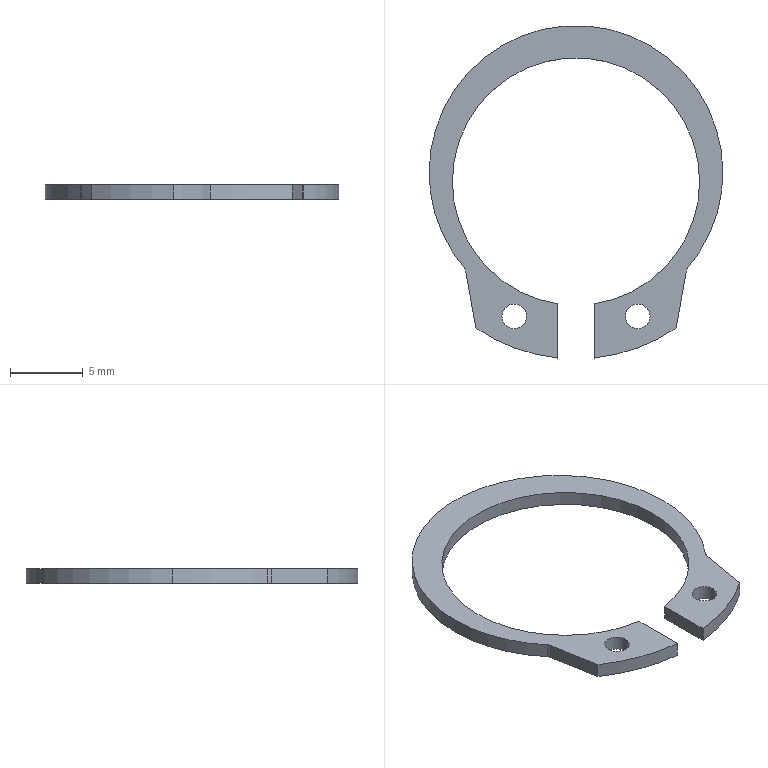Component | SolidWorks | 18A-typeShaftRetainingRing(GB-T894.1-1986)0-2 | 1 solid | 20 faces | box 20.2 x 22.86 x 1 mm | volume 122 mm3 | cylinder 14 | plane 6 | commonest cylinder face diameters 1.7 x4 20.2 x3 17 x3 24.4 x2 1 x2 | material 65Mn CH
build123d program:
from build123d import *

# Parameters (mm, degrees)
SKETCH1_R           = 0.85
BOSS_EXTRUDE1_DEPTH = 1


with BuildPart() as part:
    # Sketch1 → Boss-Extrude1 (new body)
    with BuildSketch(Plane.XY):
        with BuildLine():
            Line((-7.583, -6.16), (-6.894, -10.065))
            ThreePointArc((-6.894, -10.065), (-4.202, -11.454), (-1.25, -12.136))
            Line((-1.25, -12.136), (-1.25, -8.408))
            ThreePointArc((-1.25, -8.408), (0, 8.5), (1.25, -8.408))
            Line((1.25, -8.408), (1.25, -12.136))
            ThreePointArc((1.25, -12.136), (4.202, -11.454), (6.894, -10.065))
            Line((6.894, -10.065), (7.583, -6.16))
            ThreePointArc((7.583, -6.16), (7.623, -6.034), (7.694, -5.923))
            ThreePointArc((7.694, -5.923), (0, 10.72), (-7.694, -5.923))
            ThreePointArc((-7.694, -5.923), (-7.623, -6.034), (-7.583, -6.16))
        make_face()
        with Locations((-4.25, -9.27)):
            Circle(SKETCH1_R, mode=Mode.SUBTRACT)
        with Locations((4.25, -9.27)):
            Circle(SKETCH1_R, mode=Mode.SUBTRACT)
    extrude(amount=BOSS_EXTRUDE1_DEPTH)


solid = part.part

# Placed as in the assembly
solid = solid.moved(Location((-15.093, -37.782, 147.955), (0, 0, 0)))
STEP:
#1=COLOUR_RGB('',0.7922,0.8196,0.9333);
#2=FILL_AREA_STYLE_COLOUR('',#1);
#3=FILL_AREA_STYLE('',(#2));
#4=SURFACE_STYLE_FILL_AREA(#3);
#5=SURFACE_SIDE_STYLE('',(#4));
#6=SURFACE_STYLE_USAGE(.BOTH.,#5);
#7=PRESENTATION_STYLE_ASSIGNMENT((#6));
#8=CARTESIAN_POINT('',(-0.4604,-1.852,5.864));
#9=VERTEX_POINT('',#8);
#10=CARTESIAN_POINT('',(-0.3934,-1.852,5.864));
#11=VERTEX_POINT('',#10);
#12=CARTESIAN_POINT('',(-0.4269,-1.852,5.864));
#13=DIRECTION('',(0.,0.,1.));
#14=DIRECTION('',(1.,0.,0.));
#15=AXIS2_PLACEMENT_3D('',#12,#13,#14);
#16=CIRCLE('',#15,0.03346);
#17=EDGE_CURVE('',#9,#11,#16,.T.);
#18=ORIENTED_EDGE('',*,*,#17,.T.);
#19=CARTESIAN_POINT('',(-0.3934,-1.852,5.825));
#20=VERTEX_POINT('',#19);
#21=CARTESIAN_POINT('',(-0.3934,-1.852,5.864));
#22=DIRECTION('',(0.,0.,-1.));
#23=VECTOR('',#22,39.37);
#24=LINE('',#21,#23);
#25=EDGE_CURVE('',#11,#20,#24,.T.);
#26=ORIENTED_EDGE('',*,*,#25,.T.);
#27=CARTESIAN_POINT('',(-0.4604,-1.852,5.825));
#28=VERTEX_POINT('',#27);
#29=CARTESIAN_POINT('',(-0.4269,-1.852,5.825));
#30=DIRECTION('',(0.,0.,1.));
#31=DIRECTION('',(1.,0.,0.));
#32=AXIS2_PLACEMENT_3D('',#29,#30,#31);
#33=CIRCLE('',#32,0.03346);
#34=EDGE_CURVE('',#28,#20,#33,.T.);
#35=ORIENTED_EDGE('',*,*,#34,.F.);
#36=CARTESIAN_POINT('',(-0.4604,-1.852,5.864));
#37=DIRECTION('',(0.,0.,-1.));
#38=VECTOR('',#37,39.37);
#39=LINE('',#36,#38);
#40=EDGE_CURVE('',#9,#28,#39,.T.);
#41=ORIENTED_EDGE('',*,*,#40,.F.);
#42=EDGE_LOOP('',(#18,#26,#35,#41));
#43=FACE_OUTER_BOUND('',#42,.T.);
#44=CARTESIAN_POINT('',(-0.4269,-1.852,5.864));
#45=DIRECTION('',(0.,0.,-1.));
#46=DIRECTION('',(-1.,0.,0.));
#47=AXIS2_PLACEMENT_3D('',#44,#45,#46);
#48=CYLINDRICAL_SURFACE('',#47,0.03346);
#49=ADVANCED_FACE('',(#43),#48,.F.);
#50=CARTESIAN_POINT('',(-0.795,-1.852,5.864));
#51=VERTEX_POINT('',#50);
#52=CARTESIAN_POINT('',(-0.7281,-1.852,5.864));
#53=VERTEX_POINT('',#52);
#54=CARTESIAN_POINT('',(-0.7615,-1.852,5.864));
#55=DIRECTION('',(0.,0.,1.));
#56=DIRECTION('',(1.,0.,0.));
#57=AXIS2_PLACEMENT_3D('',#54,#55,#56);
#58=CIRCLE('',#57,0.03346);
#59=EDGE_CURVE('',#51,#53,#58,.T.);
#60=ORIENTED_EDGE('',*,*,#59,.T.);
#61=CARTESIAN_POINT('',(-0.7281,-1.852,5.825));
#62=VERTEX_POINT('',#61);
#63=CARTESIAN_POINT('',(-0.7281,-1.852,5.864));
#64=DIRECTION('',(0.,0.,-1.));
#65=VECTOR('',#64,39.37);
#66=LINE('',#63,#65);
#67=EDGE_CURVE('',#53,#62,#66,.T.);
#68=ORIENTED_EDGE('',*,*,#67,.T.);
#69=CARTESIAN_POINT('',(-0.795,-1.852,5.825));
#70=VERTEX_POINT('',#69);
#71=CARTESIAN_POINT('',(-0.7615,-1.852,5.825));
#72=DIRECTION('',(0.,0.,1.));
#73=DIRECTION('',(1.,0.,0.));
#74=AXIS2_PLACEMENT_3D('',#71,#72,#73);
#75=CIRCLE('',#74,0.03346);
#76=EDGE_CURVE('',#70,#62,#75,.T.);
#77=ORIENTED_EDGE('',*,*,#76,.F.);
#78=CARTESIAN_POINT('',(-0.795,-1.852,5.864));
#79=DIRECTION('',(0.,0.,-1.));
#80=VECTOR('',#79,39.37);
#81=LINE('',#78,#80);
#82=EDGE_CURVE('',#51,#70,#81,.T.);
#83=ORIENTED_EDGE('',*,*,#82,.F.);
#84=EDGE_LOOP('',(#60,#68,#77,#83));
#85=FACE_OUTER_BOUND('',#84,.T.);
#86=CARTESIAN_POINT('',(-0.7615,-1.852,5.864));
#87=DIRECTION('',(0.,0.,-1.));
#88=DIRECTION('',(-1.,0.,0.));
#89=AXIS2_PLACEMENT_3D('',#86,#87,#88);
#90=CYLINDRICAL_SURFACE('',#89,0.03346);
#91=ADVANCED_FACE('',(#85),#90,.F.);
#92=CARTESIAN_POINT('',(-0.1966,-1.463,5.864));
#93=VERTEX_POINT('',#92);
#94=CARTESIAN_POINT('',(-0.9919,-1.463,5.864));
#95=VERTEX_POINT('',#94);
#96=CARTESIAN_POINT('',(-0.5942,-1.463,5.864));
#97=DIRECTION('',(0.,0.,1.));
#98=DIRECTION('',(1.,0.,0.));
#99=AXIS2_PLACEMENT_3D('',#96,#97,#98);
#100=CIRCLE('',#99,0.3976);
#101=EDGE_CURVE('',#93,#95,#100,.T.);
#102=ORIENTED_EDGE('',*,*,#101,.F.);
#103=CARTESIAN_POINT('',(-0.1966,-1.463,5.825));
#104=VERTEX_POINT('',#103);
#105=CARTESIAN_POINT('',(-0.1966,-1.463,5.864));
#106=DIRECTION('',(0.,0.,-1.));
#107=VECTOR('',#106,39.37);
#108=LINE('',#105,#107);
#109=EDGE_CURVE('',#93,#104,#108,.T.);
#110=ORIENTED_EDGE('',*,*,#109,.T.);
#111=CARTESIAN_POINT('',(-0.9919,-1.463,5.825));
#112=VERTEX_POINT('',#111);
#113=CARTESIAN_POINT('',(-0.5942,-1.463,5.825));
#114=DIRECTION('',(0.,0.,1.));
#115=DIRECTION('',(1.,0.,0.));
#116=AXIS2_PLACEMENT_3D('',#113,#114,#115);
#117=CIRCLE('',#116,0.3976);
#118=EDGE_CURVE('',#104,#112,#117,.T.);
#119=ORIENTED_EDGE('',*,*,#118,.T.);
#120=CARTESIAN_POINT('',(-0.9919,-1.463,5.864));
#121=DIRECTION('',(0.,0.,-1.));
#122=VECTOR('',#121,39.37);
#123=LINE('',#120,#122);
#124=EDGE_CURVE('',#95,#112,#123,.T.);
#125=ORIENTED_EDGE('',*,*,#124,.F.);
#126=EDGE_LOOP('',(#102,#110,#119,#125));
#127=FACE_OUTER_BOUND('',#126,.T.);
#128=CARTESIAN_POINT('',(-0.5942,-1.463,5.864));
#129=DIRECTION('',(0.,0.,-1.));
#130=DIRECTION('',(-1.,0.,0.));
#131=AXIS2_PLACEMENT_3D('',#128,#129,#130);
#132=CYLINDRICAL_SURFACE('',#131,0.3976);
#133=ADVANCED_FACE('',(#127),#132,.T.);
#134=CARTESIAN_POINT('',(-0.8971,-1.721,5.864));
#135=VERTEX_POINT('',#134);
#136=CARTESIAN_POINT('',(-0.5942,-1.463,5.864));
#137=DIRECTION('',(0.,0.,1.));
#138=DIRECTION('',(1.,0.,0.));
#139=AXIS2_PLACEMENT_3D('',#136,#137,#138);
#140=CIRCLE('',#139,0.3976);
#141=EDGE_CURVE('',#95,#135,#140,.T.);
#142=ORIENTED_EDGE('',*,*,#141,.F.);
#143=ORIENTED_EDGE('',*,*,#124,.T.);
#144=CARTESIAN_POINT('',(-0.8971,-1.721,5.825));
#145=VERTEX_POINT('',#144);
#146=CARTESIAN_POINT('',(-0.5942,-1.463,5.825));
#147=DIRECTION('',(0.,0.,1.));
#148=DIRECTION('',(1.,0.,0.));
#149=AXIS2_PLACEMENT_3D('',#146,#147,#148);
#150=CIRCLE('',#149,0.3976);
#151=EDGE_CURVE('',#112,#145,#150,.T.);
#152=ORIENTED_EDGE('',*,*,#151,.T.);
#153=CARTESIAN_POINT('',(-0.8971,-1.721,5.864));
#154=DIRECTION('',(0.,0.,-1.));
#155=VECTOR('',#154,39.37);
#156=LINE('',#153,#155);
#157=EDGE_CURVE('',#135,#145,#156,.T.);
#158=ORIENTED_EDGE('',*,*,#157,.F.);
#159=EDGE_LOOP('',(#142,#143,#152,#158));
#160=FACE_OUTER_BOUND('',#159,.T.);
#161=CARTESIAN_POINT('',(-0.5942,-1.463,5.864));
#162=DIRECTION('',(0.,0.,-1.));
#163=DIRECTION('',(-1.,0.,0.));
#164=AXIS2_PLACEMENT_3D('',#161,#162,#163);
#165=CYLINDRICAL_SURFACE('',#164,0.3976);
#166=ADVANCED_FACE('',(#160),#165,.T.);
#167=CARTESIAN_POINT('',(-0.2596,-1.487,5.864));
#168=VERTEX_POINT('',#167);
#169=CARTESIAN_POINT('',(-0.545,-1.818,5.864));
#170=VERTEX_POINT('',#169);
#171=CARTESIAN_POINT('',(-0.5942,-1.487,5.864));
#172=DIRECTION('',(0.,0.,-1.));
#173=DIRECTION('',(1.,0.,0.));
#174=AXIS2_PLACEMENT_3D('',#171,#172,#173);
#175=CIRCLE('',#174,0.3346);
#176=EDGE_CURVE('',#168,#170,#175,.T.);
#177=ORIENTED_EDGE('',*,*,#176,.F.);
#178=CARTESIAN_POINT('',(-0.2596,-1.487,5.825));
#179=VERTEX_POINT('',#178);
#180=CARTESIAN_POINT('',(-0.2596,-1.487,5.864));
#181=DIRECTION('',(0.,0.,-1.));
#182=VECTOR('',#181,39.37);
#183=LINE('',#180,#182);
#184=EDGE_CURVE('',#168,#179,#183,.T.);
#185=ORIENTED_EDGE('',*,*,#184,.T.);
#186=CARTESIAN_POINT('',(-0.545,-1.818,5.825));
#187=VERTEX_POINT('',#186);
#188=CARTESIAN_POINT('',(-0.5942,-1.487,5.825));
#189=DIRECTION('',(0.,0.,-1.));
#190=DIRECTION('',(1.,0.,0.));
#191=AXIS2_PLACEMENT_3D('',#188,#189,#190);
#192=CIRCLE('',#191,0.3346);
#193=EDGE_CURVE('',#179,#187,#192,.T.);
#194=ORIENTED_EDGE('',*,*,#193,.T.);
#195=CARTESIAN_POINT('',(-0.545,-1.818,5.864));
#196=DIRECTION('',(0.,0.,-1.));
#197=VECTOR('',#196,39.37);
#198=LINE('',#195,#197);
#199=EDGE_CURVE('',#170,#187,#198,.T.);
#200=ORIENTED_EDGE('',*,*,#199,.F.);
#201=EDGE_LOOP('',(#177,#185,#194,#200));
#202=FACE_OUTER_BOUND('',#201,.T.);
#203=CARTESIAN_POINT('',(-0.5942,-1.487,5.864));
#204=DIRECTION('',(0.,0.,-1.));
#205=DIRECTION('',(-1.,0.,0.));
#206=AXIS2_PLACEMENT_3D('',#203,#204,#205);
#207=CYLINDRICAL_SURFACE('',#206,0.3346);
#208=ADVANCED_FACE('',(#202),#207,.F.);
#209=ORIENTED_EDGE('',*,*,#184,.F.);
#210=CARTESIAN_POINT('',(-0.9289,-1.487,5.864));
#211=VERTEX_POINT('',#210);
#212=CARTESIAN_POINT('',(-0.5942,-1.487,5.864));
#213=DIRECTION('',(0.,0.,-1.));
#214=DIRECTION('',(1.,0.,0.));
#215=AXIS2_PLACEMENT_3D('',#212,#213,#214);
#216=CIRCLE('',#215,0.3346);
#217=EDGE_CURVE('',#211,#168,#216,.T.);
#218=ORIENTED_EDGE('',*,*,#217,.F.);
#219=CARTESIAN_POINT('',(-0.9289,-1.487,5.825));
#220=VERTEX_POINT('',#219);
#221=CARTESIAN_POINT('',(-0.9289,-1.487,5.864));
#222=DIRECTION('',(0.,0.,-1.));
#223=VECTOR('',#222,39.37);
#224=LINE('',#221,#223);
#225=EDGE_CURVE('',#211,#220,#224,.T.);
#226=ORIENTED_EDGE('',*,*,#225,.T.);
#227=CARTESIAN_POINT('',(-0.5942,-1.487,5.825));
#228=DIRECTION('',(0.,0.,-1.));
#229=DIRECTION('',(1.,0.,0.));
#230=AXIS2_PLACEMENT_3D('',#227,#228,#229);
#231=CIRCLE('',#230,0.3346);
#232=EDGE_CURVE('',#220,#179,#231,.T.);
#233=ORIENTED_EDGE('',*,*,#232,.T.);
#234=EDGE_LOOP('',(#209,#218,#226,#233));
#235=FACE_OUTER_BOUND('',#234,.T.);
#236=CARTESIAN_POINT('',(-0.5942,-1.487,5.864));
#237=DIRECTION('',(0.,0.,-1.));
#238=DIRECTION('',(-1.,0.,0.));
#239=AXIS2_PLACEMENT_3D('',#236,#237,#238);
#240=CYLINDRICAL_SURFACE('',#239,0.3346);
#241=ADVANCED_FACE('',(#235),#240,.F.);
#242=ORIENTED_EDGE('',*,*,#59,.F.);
#243=CARTESIAN_POINT('',(-0.7615,-1.852,5.864));
#244=DIRECTION('',(0.,0.,1.));
#245=DIRECTION('',(1.,0.,0.));
#246=AXIS2_PLACEMENT_3D('',#243,#244,#245);
#247=CIRCLE('',#246,0.03346);
#248=EDGE_CURVE('',#53,#51,#247,.T.);
#249=ORIENTED_EDGE('',*,*,#248,.F.);
#250=EDGE_LOOP('',(#242,#249));
#251=FACE_BOUND('',#250,.T.);
#252=CARTESIAN_POINT('',(-0.6434,-1.818,5.864));
#253=VERTEX_POINT('',#252);
#254=CARTESIAN_POINT('',(-0.5942,-1.487,5.864));
#255=DIRECTION('',(0.,0.,-1.));
#256=DIRECTION('',(1.,0.,0.));
#257=AXIS2_PLACEMENT_3D('',#254,#255,#256);
#258=CIRCLE('',#257,0.3346);
#259=EDGE_CURVE('',#253,#211,#258,.T.);
#260=ORIENTED_EDGE('',*,*,#259,.T.);
#261=ORIENTED_EDGE('',*,*,#217,.T.);
#262=ORIENTED_EDGE('',*,*,#176,.T.);
#263=CARTESIAN_POINT('',(-0.545,-1.965,5.864));
#264=VERTEX_POINT('',#263);
#265=CARTESIAN_POINT('',(-0.545,-1.818,5.864));
#266=DIRECTION('',(0.,-1.,0.));
#267=VECTOR('',#266,39.37);
#268=LINE('',#265,#267);
#269=EDGE_CURVE('',#170,#264,#268,.T.);
#270=ORIENTED_EDGE('',*,*,#269,.T.);
#271=CARTESIAN_POINT('',(-0.3228,-1.884,5.864));
#272=VERTEX_POINT('',#271);
#273=CARTESIAN_POINT('',(-0.5942,-1.487,5.864));
#274=DIRECTION('',(0.,0.,1.));
#275=DIRECTION('',(1.,0.,0.));
#276=AXIS2_PLACEMENT_3D('',#273,#274,#275);
#277=CIRCLE('',#276,0.4803);
#278=EDGE_CURVE('',#264,#272,#277,.T.);
#279=ORIENTED_EDGE('',*,*,#278,.T.);
#280=CARTESIAN_POINT('',(-0.2957,-1.73,5.864));
#281=VERTEX_POINT('',#280);
#282=CARTESIAN_POINT('',(-0.2957,-1.73,5.864));
#283=DIRECTION('',(0.1736,0.9848,0.));
#284=VECTOR('',#283,39.37);
#285=LINE('',#282,#284);
#286=EDGE_CURVE('',#272,#281,#285,.T.);
#287=ORIENTED_EDGE('',*,*,#286,.T.);
#288=CARTESIAN_POINT('',(-0.2913,-1.721,5.864));
#289=VERTEX_POINT('',#288);
#290=CARTESIAN_POINT('',(-0.2763,-1.733,5.864));
#291=DIRECTION('',(0.,0.,-1.));
#292=DIRECTION('',(1.,0.,0.));
#293=AXIS2_PLACEMENT_3D('',#290,#291,#292);
#294=CIRCLE('',#293,0.01969);
#295=EDGE_CURVE('',#281,#289,#294,.T.);
#296=ORIENTED_EDGE('',*,*,#295,.T.);
#297=CARTESIAN_POINT('',(-0.5942,-1.463,5.864));
#298=DIRECTION('',(0.,0.,1.));
#299=DIRECTION('',(1.,0.,0.));
#300=AXIS2_PLACEMENT_3D('',#297,#298,#299);
#301=CIRCLE('',#300,0.3976);
#302=EDGE_CURVE('',#289,#93,#301,.T.);
#303=ORIENTED_EDGE('',*,*,#302,.T.);
#304=ORIENTED_EDGE('',*,*,#101,.T.);
#305=ORIENTED_EDGE('',*,*,#141,.T.);
#306=CARTESIAN_POINT('',(-0.8927,-1.73,5.864));
#307=VERTEX_POINT('',#306);
#308=CARTESIAN_POINT('',(-0.9121,-1.733,5.864));
#309=DIRECTION('',(0.,0.,-1.));
#310=DIRECTION('',(1.,0.,0.));
#311=AXIS2_PLACEMENT_3D('',#308,#309,#310);
#312=CIRCLE('',#311,0.01969);
#313=EDGE_CURVE('',#135,#307,#312,.T.);
#314=ORIENTED_EDGE('',*,*,#313,.T.);
#315=CARTESIAN_POINT('',(-0.8656,-1.884,5.864));
#316=VERTEX_POINT('',#315);
#317=CARTESIAN_POINT('',(-0.8927,-1.73,5.864));
#318=DIRECTION('',(0.1736,-0.9848,0.));
#319=VECTOR('',#318,39.37);
#320=LINE('',#317,#319);
#321=EDGE_CURVE('',#307,#316,#320,.T.);
#322=ORIENTED_EDGE('',*,*,#321,.T.);
#323=CARTESIAN_POINT('',(-0.6434,-1.965,5.864));
#324=VERTEX_POINT('',#323);
#325=CARTESIAN_POINT('',(-0.5942,-1.487,5.864));
#326=DIRECTION('',(0.,0.,1.));
#327=DIRECTION('',(1.,0.,0.));
#328=AXIS2_PLACEMENT_3D('',#325,#326,#327);
#329=CIRCLE('',#328,0.4803);
#330=EDGE_CURVE('',#316,#324,#329,.T.);
#331=ORIENTED_EDGE('',*,*,#330,.T.);
#332=CARTESIAN_POINT('',(-0.6434,-1.818,5.864));
#333=DIRECTION('',(0.,1.,0.));
#334=VECTOR('',#333,39.37);
#335=LINE('',#332,#334);
#336=EDGE_CURVE('',#324,#253,#335,.T.);
#337=ORIENTED_EDGE('',*,*,#336,.T.);
#338=EDGE_LOOP('',(#260,#261,#262,#270,#279,#287,#296,#303,#304,#305,#314,#322,#331,#337));
#339=FACE_OUTER_BOUND('',#338,.T.);
#340=ORIENTED_EDGE('',*,*,#17,.F.);
#341=CARTESIAN_POINT('',(-0.4269,-1.852,5.864));
#342=DIRECTION('',(0.,0.,1.));
#343=DIRECTION('',(1.,0.,0.));
#344=AXIS2_PLACEMENT_3D('',#341,#342,#343);
#345=CIRCLE('',#344,0.03346);
#346=EDGE_CURVE('',#11,#9,#345,.T.);
#347=ORIENTED_EDGE('',*,*,#346,.F.);
#348=EDGE_LOOP('',(#340,#347));
#349=FACE_BOUND('',#348,.T.);
#350=CARTESIAN_POINT('',(-0.5942,-1.487,5.864));
#351=DIRECTION('',(0.,0.,1.));
#352=DIRECTION('',(1.,0.,0.));
#353=AXIS2_PLACEMENT_3D('',#350,#351,#352);
#354=PLANE('',#353);
#355=ADVANCED_FACE('',(#251,#339,#349),#354,.T.);
#356=CARTESIAN_POINT('',(-0.6434,-1.818,5.825));
#357=VERTEX_POINT('',#356);
#358=CARTESIAN_POINT('',(-0.5942,-1.487,5.825));
#359=DIRECTION('',(0.,0.,-1.));
#360=DIRECTION('',(1.,0.,0.));
#361=AXIS2_PLACEMENT_3D('',#358,#359,#360);
#362=CIRCLE('',#361,0.3346);
#363=EDGE_CURVE('',#357,#220,#362,.T.);
#364=ORIENTED_EDGE('',*,*,#363,.F.);
#365=CARTESIAN_POINT('',(-0.6434,-1.965,5.825));
#366=VERTEX_POINT('',#365);
#367=CARTESIAN_POINT('',(-0.6434,-1.818,5.825));
#368=DIRECTION('',(0.,1.,0.));
#369=VECTOR('',#368,39.37);
#370=LINE('',#367,#369);
#371=EDGE_CURVE('',#366,#357,#370,.T.);
#372=ORIENTED_EDGE('',*,*,#371,.F.);
#373=CARTESIAN_POINT('',(-0.8656,-1.884,5.825));
#374=VERTEX_POINT('',#373);
#375=CARTESIAN_POINT('',(-0.5942,-1.487,5.825));
#376=DIRECTION('',(0.,0.,1.));
#377=DIRECTION('',(1.,0.,0.));
#378=AXIS2_PLACEMENT_3D('',#375,#376,#377);
#379=CIRCLE('',#378,0.4803);
#380=EDGE_CURVE('',#374,#366,#379,.T.);
#381=ORIENTED_EDGE('',*,*,#380,.F.);
#382=CARTESIAN_POINT('',(-0.8927,-1.73,5.825));
#383=VERTEX_POINT('',#382);
#384=CARTESIAN_POINT('',(-0.8927,-1.73,5.825));
#385=DIRECTION('',(0.1736,-0.9848,0.));
#386=VECTOR('',#385,39.37);
#387=LINE('',#384,#386);
#388=EDGE_CURVE('',#383,#374,#387,.T.);
#389=ORIENTED_EDGE('',*,*,#388,.F.);
#390=CARTESIAN_POINT('',(-0.9121,-1.733,5.825));
#391=DIRECTION('',(0.,0.,-1.));
#392=DIRECTION('',(1.,0.,0.));
#393=AXIS2_PLACEMENT_3D('',#390,#391,#392);
#394=CIRCLE('',#393,0.01969);
#395=EDGE_CURVE('',#145,#383,#394,.T.);
#396=ORIENTED_EDGE('',*,*,#395,.F.);
#397=ORIENTED_EDGE('',*,*,#151,.F.);
#398=ORIENTED_EDGE('',*,*,#118,.F.);
#399=CARTESIAN_POINT('',(-0.2913,-1.721,5.825));
#400=VERTEX_POINT('',#399);
#401=CARTESIAN_POINT('',(-0.5942,-1.463,5.825));
#402=DIRECTION('',(0.,0.,1.));
#403=DIRECTION('',(1.,0.,0.));
#404=AXIS2_PLACEMENT_3D('',#401,#402,#403);
#405=CIRCLE('',#404,0.3976);
#406=EDGE_CURVE('',#400,#104,#405,.T.);
#407=ORIENTED_EDGE('',*,*,#406,.F.);
#408=CARTESIAN_POINT('',(-0.2957,-1.73,5.825));
#409=VERTEX_POINT('',#408);
#410=CARTESIAN_POINT('',(-0.2763,-1.733,5.825));
#411=DIRECTION('',(0.,0.,-1.));
#412=DIRECTION('',(1.,0.,0.));
#413=AXIS2_PLACEMENT_3D('',#410,#411,#412);
#414=CIRCLE('',#413,0.01969);
#415=EDGE_CURVE('',#409,#400,#414,.T.);
#416=ORIENTED_EDGE('',*,*,#415,.F.);
#417=CARTESIAN_POINT('',(-0.3228,-1.884,5.825));
#418=VERTEX_POINT('',#417);
#419=CARTESIAN_POINT('',(-0.2957,-1.73,5.825));
#420=DIRECTION('',(0.1736,0.9848,0.));
#421=VECTOR('',#420,39.37);
#422=LINE('',#419,#421);
#423=EDGE_CURVE('',#418,#409,#422,.T.);
#424=ORIENTED_EDGE('',*,*,#423,.F.);
#425=CARTESIAN_POINT('',(-0.545,-1.965,5.825));
#426=VERTEX_POINT('',#425);
#427=CARTESIAN_POINT('',(-0.5942,-1.487,5.825));
#428=DIRECTION('',(0.,0.,1.));
#429=DIRECTION('',(1.,0.,0.));
#430=AXIS2_PLACEMENT_3D('',#427,#428,#429);
#431=CIRCLE('',#430,0.4803);
#432=EDGE_CURVE('',#426,#418,#431,.T.);
#433=ORIENTED_EDGE('',*,*,#432,.F.);
#434=CARTESIAN_POINT('',(-0.545,-1.818,5.825));
#435=DIRECTION('',(0.,-1.,0.));
#436=VECTOR('',#435,39.37);
#437=LINE('',#434,#436);
#438=EDGE_CURVE('',#187,#426,#437,.T.);
#439=ORIENTED_EDGE('',*,*,#438,.F.);
#440=ORIENTED_EDGE('',*,*,#193,.F.);
#441=ORIENTED_EDGE('',*,*,#232,.F.);
#442=EDGE_LOOP('',(#364,#372,#381,#389,#396,#397,#398,#407,#416,#424,#433,#439,#440,#441));
#443=FACE_OUTER_BOUND('',#442,.T.);
#444=ORIENTED_EDGE('',*,*,#76,.T.);
#445=CARTESIAN_POINT('',(-0.7615,-1.852,5.825));
#446=DIRECTION('',(0.,0.,1.));
#447=DIRECTION('',(1.,0.,0.));
#448=AXIS2_PLACEMENT_3D('',#445,#446,#447);
#449=CIRCLE('',#448,0.03346);
#450=EDGE_CURVE('',#62,#70,#449,.T.);
#451=ORIENTED_EDGE('',*,*,#450,.T.);
#452=EDGE_LOOP('',(#444,#451));
#453=FACE_BOUND('',#452,.T.);
#454=ORIENTED_EDGE('',*,*,#34,.T.);
#455=CARTESIAN_POINT('',(-0.4269,-1.852,5.825));
#456=DIRECTION('',(0.,0.,1.));
#457=DIRECTION('',(1.,0.,0.));
#458=AXIS2_PLACEMENT_3D('',#455,#456,#457);
#459=CIRCLE('',#458,0.03346);
#460=EDGE_CURVE('',#20,#28,#459,.T.);
#461=ORIENTED_EDGE('',*,*,#460,.T.);
#462=EDGE_LOOP('',(#454,#461));
#463=FACE_BOUND('',#462,.T.);
#464=CARTESIAN_POINT('',(-0.5942,-1.487,5.825));
#465=DIRECTION('',(0.,0.,1.));
#466=DIRECTION('',(1.,0.,0.));
#467=AXIS2_PLACEMENT_3D('',#464,#465,#466);
#468=PLANE('',#467);
#469=ADVANCED_FACE('',(#443,#453,#463),#468,.F.);
#470=ORIENTED_EDGE('',*,*,#225,.F.);
#471=ORIENTED_EDGE('',*,*,#259,.F.);
#472=CARTESIAN_POINT('',(-0.6434,-1.818,5.864));
#473=DIRECTION('',(0.,0.,-1.));
#474=VECTOR('',#473,39.37);
#475=LINE('',#472,#474);
#476=EDGE_CURVE('',#253,#357,#475,.T.);
#477=ORIENTED_EDGE('',*,*,#476,.T.);
#478=ORIENTED_EDGE('',*,*,#363,.T.);
#479=EDGE_LOOP('',(#470,#471,#477,#478));
#480=FACE_OUTER_BOUND('',#479,.T.);
#481=CARTESIAN_POINT('',(-0.5942,-1.487,5.864));
#482=DIRECTION('',(0.,0.,-1.));
#483=DIRECTION('',(-1.,0.,0.));
#484=AXIS2_PLACEMENT_3D('',#481,#482,#483);
#485=CYLINDRICAL_SURFACE('',#484,0.3346);
#486=ADVANCED_FACE('',(#480),#485,.F.);
#487=ORIENTED_EDGE('',*,*,#438,.T.);
#488=CARTESIAN_POINT('',(-0.545,-1.965,5.864));
#489=DIRECTION('',(0.,0.,-1.));
#490=VECTOR('',#489,39.37);
#491=LINE('',#488,#490);
#492=EDGE_CURVE('',#264,#426,#491,.T.);
#493=ORIENTED_EDGE('',*,*,#492,.F.);
#494=ORIENTED_EDGE('',*,*,#269,.F.);
#495=ORIENTED_EDGE('',*,*,#199,.T.);
#496=EDGE_LOOP('',(#487,#493,#494,#495));
#497=FACE_OUTER_BOUND('',#496,.T.);
#498=CARTESIAN_POINT('',(-0.545,-1.818,5.864));
#499=DIRECTION('',(1.,0.,0.));
#500=DIRECTION('',(0.,0.,-1.));
#501=AXIS2_PLACEMENT_3D('',#498,#499,#500);
#502=PLANE('',#501);
#503=ADVANCED_FACE('',(#497),#502,.F.);
#504=ORIENTED_EDGE('',*,*,#432,.T.);
#505=CARTESIAN_POINT('',(-0.3228,-1.884,5.864));
#506=DIRECTION('',(0.,0.,-1.));
#507=VECTOR('',#506,39.37);
#508=LINE('',#505,#507);
#509=EDGE_CURVE('',#272,#418,#508,.T.);
#510=ORIENTED_EDGE('',*,*,#509,.F.);
#511=ORIENTED_EDGE('',*,*,#278,.F.);
#512=ORIENTED_EDGE('',*,*,#492,.T.);
#513=EDGE_LOOP('',(#504,#510,#511,#512));
#514=FACE_OUTER_BOUND('',#513,.T.);
#515=CARTESIAN_POINT('',(-0.5942,-1.487,5.864));
#516=DIRECTION('',(0.,0.,-1.));
#517=DIRECTION('',(-1.,0.,0.));
#518=AXIS2_PLACEMENT_3D('',#515,#516,#517);
#519=CYLINDRICAL_SURFACE('',#518,0.4803);
#520=ADVANCED_FACE('',(#514),#519,.T.);
#521=ORIENTED_EDGE('',*,*,#423,.T.);
#522=CARTESIAN_POINT('',(-0.2957,-1.73,5.864));
#523=DIRECTION('',(0.,0.,-1.));
#524=VECTOR('',#523,39.37);
#525=LINE('',#522,#524);
#526=EDGE_CURVE('',#281,#409,#525,.T.);
#527=ORIENTED_EDGE('',*,*,#526,.F.);
#528=ORIENTED_EDGE('',*,*,#286,.F.);
#529=ORIENTED_EDGE('',*,*,#509,.T.);
#530=EDGE_LOOP('',(#521,#527,#528,#529));
#531=FACE_OUTER_BOUND('',#530,.T.);
#532=CARTESIAN_POINT('',(-0.2957,-1.73,5.864));
#533=DIRECTION('',(-0.9848,0.1736,0.));
#534=DIRECTION('',(-0.1736,-0.9848,0.));
#535=AXIS2_PLACEMENT_3D('',#532,#533,#534);
#536=PLANE('',#535);
#537=ADVANCED_FACE('',(#531),#536,.F.);
#538=ORIENTED_EDGE('',*,*,#415,.T.);
#539=CARTESIAN_POINT('',(-0.2913,-1.721,5.864));
#540=DIRECTION('',(0.,0.,-1.));
#541=VECTOR('',#540,39.37);
#542=LINE('',#539,#541);
#543=EDGE_CURVE('',#289,#400,#542,.T.);
#544=ORIENTED_EDGE('',*,*,#543,.F.);
#545=ORIENTED_EDGE('',*,*,#295,.F.);
#546=ORIENTED_EDGE('',*,*,#526,.T.);
#547=EDGE_LOOP('',(#538,#544,#545,#546));
#548=FACE_OUTER_BOUND('',#547,.T.);
#549=CARTESIAN_POINT('',(-0.2763,-1.733,5.864));
#550=DIRECTION('',(0.,0.,-1.));
#551=DIRECTION('',(-1.,0.,0.));
#552=AXIS2_PLACEMENT_3D('',#549,#550,#551);
#553=CYLINDRICAL_SURFACE('',#552,0.01969);
#554=ADVANCED_FACE('',(#548),#553,.F.);
#555=ORIENTED_EDGE('',*,*,#109,.F.);
#556=ORIENTED_EDGE('',*,*,#302,.F.);
#557=ORIENTED_EDGE('',*,*,#543,.T.);
#558=ORIENTED_EDGE('',*,*,#406,.T.);
#559=EDGE_LOOP('',(#555,#556,#557,#558));
#560=FACE_OUTER_BOUND('',#559,.T.);
#561=CARTESIAN_POINT('',(-0.5942,-1.463,5.864));
#562=DIRECTION('',(0.,0.,-1.));
#563=DIRECTION('',(-1.,0.,0.));
#564=AXIS2_PLACEMENT_3D('',#561,#562,#563);
#565=CYLINDRICAL_SURFACE('',#564,0.3976);
#566=ADVANCED_FACE('',(#560),#565,.T.);
#567=ORIENTED_EDGE('',*,*,#395,.T.);
#568=CARTESIAN_POINT('',(-0.8927,-1.73,5.864));
#569=DIRECTION('',(0.,0.,-1.));
#570=VECTOR('',#569,39.37);
#571=LINE('',#568,#570);
#572=EDGE_CURVE('',#307,#383,#571,.T.);
#573=ORIENTED_EDGE('',*,*,#572,.F.);
#574=ORIENTED_EDGE('',*,*,#313,.F.);
#575=ORIENTED_EDGE('',*,*,#157,.T.);
#576=EDGE_LOOP('',(#567,#573,#574,#575));
#577=FACE_OUTER_BOUND('',#576,.T.);
#578=CARTESIAN_POINT('',(-0.9121,-1.733,5.864));
#579=DIRECTION('',(0.,0.,-1.));
#580=DIRECTION('',(-1.,0.,0.));
#581=AXIS2_PLACEMENT_3D('',#578,#579,#580);
#582=CYLINDRICAL_SURFACE('',#581,0.01969);
#583=ADVANCED_FACE('',(#577),#582,.F.);
#584=ORIENTED_EDGE('',*,*,#388,.T.);
#585=CARTESIAN_POINT('',(-0.8656,-1.884,5.864));
#586=DIRECTION('',(0.,0.,-1.));
#587=VECTOR('',#586,39.37);
#588=LINE('',#585,#587);
#589=EDGE_CURVE('',#316,#374,#588,.T.);
#590=ORIENTED_EDGE('',*,*,#589,.F.);
#591=ORIENTED_EDGE('',*,*,#321,.F.);
#592=ORIENTED_EDGE('',*,*,#572,.T.);
#593=EDGE_LOOP('',(#584,#590,#591,#592));
#594=FACE_OUTER_BOUND('',#593,.T.);
#595=CARTESIAN_POINT('',(-0.8927,-1.73,5.864));
#596=DIRECTION('',(0.9848,0.1736,0.));
#597=DIRECTION('',(-0.1736,0.9848,0.));
#598=AXIS2_PLACEMENT_3D('',#595,#596,#597);
#599=PLANE('',#598);
#600=ADVANCED_FACE('',(#594),#599,.F.);
#601=ORIENTED_EDGE('',*,*,#380,.T.);
#602=CARTESIAN_POINT('',(-0.6434,-1.965,5.864));
#603=DIRECTION('',(0.,0.,-1.));
#604=VECTOR('',#603,39.37);
#605=LINE('',#602,#604);
#606=EDGE_CURVE('',#324,#366,#605,.T.);
#607=ORIENTED_EDGE('',*,*,#606,.F.);
#608=ORIENTED_EDGE('',*,*,#330,.F.);
#609=ORIENTED_EDGE('',*,*,#589,.T.);
#610=EDGE_LOOP('',(#601,#607,#608,#609));
#611=FACE_OUTER_BOUND('',#610,.T.);
#612=CARTESIAN_POINT('',(-0.5942,-1.487,5.864));
#613=DIRECTION('',(0.,0.,-1.));
#614=DIRECTION('',(-1.,0.,0.));
#615=AXIS2_PLACEMENT_3D('',#612,#613,#614);
#616=CYLINDRICAL_SURFACE('',#615,0.4803);
#617=ADVANCED_FACE('',(#611),#616,.T.);
#618=ORIENTED_EDGE('',*,*,#371,.T.);
#619=ORIENTED_EDGE('',*,*,#476,.F.);
#620=ORIENTED_EDGE('',*,*,#336,.F.);
#621=ORIENTED_EDGE('',*,*,#606,.T.);
#622=EDGE_LOOP('',(#618,#619,#620,#621));
#623=FACE_OUTER_BOUND('',#622,.T.);
#624=CARTESIAN_POINT('',(-0.6434,-1.818,5.864));
#625=DIRECTION('',(-1.,0.,0.));
#626=DIRECTION('',(0.,0.,1.));
#627=AXIS2_PLACEMENT_3D('',#624,#625,#626);
#628=PLANE('',#627);
#629=ADVANCED_FACE('',(#623),#628,.F.);
#630=ORIENTED_EDGE('',*,*,#67,.F.);
#631=ORIENTED_EDGE('',*,*,#248,.T.);
#632=ORIENTED_EDGE('',*,*,#82,.T.);
#633=ORIENTED_EDGE('',*,*,#450,.F.);
#634=EDGE_LOOP('',(#630,#631,#632,#633));
#635=FACE_OUTER_BOUND('',#634,.T.);
#636=CARTESIAN_POINT('',(-0.7615,-1.852,5.864));
#637=DIRECTION('',(0.,0.,-1.));
#638=DIRECTION('',(-1.,0.,0.));
#639=AXIS2_PLACEMENT_3D('',#636,#637,#638);
#640=CYLINDRICAL_SURFACE('',#639,0.03346);
#641=ADVANCED_FACE('',(#635),#640,.F.);
#642=ORIENTED_EDGE('',*,*,#25,.F.);
#643=ORIENTED_EDGE('',*,*,#346,.T.);
#644=ORIENTED_EDGE('',*,*,#40,.T.);
#645=ORIENTED_EDGE('',*,*,#460,.F.);
#646=EDGE_LOOP('',(#642,#643,#644,#645));
#647=FACE_OUTER_BOUND('',#646,.T.);
#648=CARTESIAN_POINT('',(-0.4269,-1.852,5.864));
#649=DIRECTION('',(0.,0.,-1.));
#650=DIRECTION('',(-1.,0.,0.));
#651=AXIS2_PLACEMENT_3D('',#648,#649,#650);
#652=CYLINDRICAL_SURFACE('',#651,0.03346);
#653=ADVANCED_FACE('',(#647),#652,.F.);
#654=CLOSED_SHELL('',(#49,#91,#133,#166,#208,#241,#355,#469,#486,#503,#520,#537,#554,#566,#583,#600,#617,#629,#641,#653));
#655=MANIFOLD_SOLID_BREP('',#654);
#656=STYLED_ITEM('',(#7),#655);
#657=PRESENTATION_LAYER_ASSIGNMENT('','',(#656));
#658=CARTESIAN_POINT('',(0.,0.,0.));
#659=DIRECTION('',(0.,0.,1.));
#660=DIRECTION('',(1.,0.,0.));
#661=AXIS2_PLACEMENT_3D('',#658,#659,#660);
#662=(LENGTH_UNIT()NAMED_UNIT(*)SI_UNIT($,.METRE.));
#663=LENGTH_MEASURE_WITH_UNIT(LENGTH_MEASURE(0.0254),#662);
#664=DIMENSIONAL_EXPONENTS(1.,0.,0.,0.,0.,0.,0.);
#665=(CONVERSION_BASED_UNIT('',#663)LENGTH_UNIT()NAMED_UNIT(#664));
#666=UNCERTAINTY_MEASURE_WITH_UNIT(LENGTH_MEASURE(0.00001),#665,'','');
#667=(NAMED_UNIT(*)PLANE_ANGLE_UNIT()SI_UNIT($,.RADIAN.));
#668=(NAMED_UNIT(*)SI_UNIT($,.STERADIAN.)SOLID_ANGLE_UNIT());
#669=(GEOMETRIC_REPRESENTATION_CONTEXT(3)GLOBAL_UNCERTAINTY_ASSIGNED_CONTEXT((#666))GLOBAL_UNIT_ASSIGNED_CONTEXT((#665,#667,#668))REPRESENTATION_CONTEXT('',''));
#670=ADVANCED_BREP_SHAPE_REPRESENTATION('',(#655,#661),#669);
#671=(LENGTH_UNIT()NAMED_UNIT(*)SI_UNIT($,.METRE.));
#672=LENGTH_MEASURE_WITH_UNIT(LENGTH_MEASURE(0.0254),#671);
#673=DIMENSIONAL_EXPONENTS(1.,0.,0.,0.,0.,0.,0.);
#674=(CONVERSION_BASED_UNIT('',#672)LENGTH_UNIT()NAMED_UNIT(#673));
#675=UNCERTAINTY_MEASURE_WITH_UNIT(LENGTH_MEASURE(0.00001),#674,'','');
#676=(NAMED_UNIT(*)PLANE_ANGLE_UNIT()SI_UNIT($,.RADIAN.));
#677=(NAMED_UNIT(*)SI_UNIT($,.STERADIAN.)SOLID_ANGLE_UNIT());
#678=(GEOMETRIC_REPRESENTATION_CONTEXT(3)GLOBAL_UNCERTAINTY_ASSIGNED_CONTEXT((#675))GLOBAL_UNIT_ASSIGNED_CONTEXT((#674,#676,#677))REPRESENTATION_CONTEXT('',''));
#679=MECHANICAL_DESIGN_GEOMETRIC_PRESENTATION_REPRESENTATION('',(#656),#678);